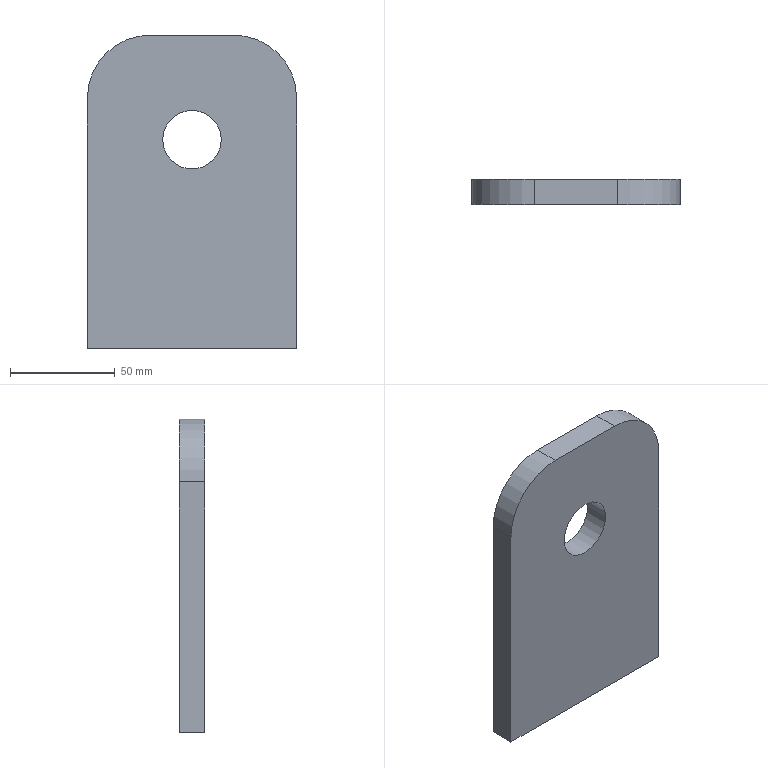Component | NX | CHAPA_GARAFA_2 | 1 solid | 9 faces | box 100 x 12 x 150 mm | volume 167976 mm3 | plane 6 | cylinder 3 | commonest cylinder face diameters 60 x2 28 x1
STEP:
#1=CARTESIAN_POINT('',(0.,0.,0.));
#2=DIRECTION('',(0.,0.,1.));
#3=DIRECTION('',(1.,0.,0.));
#4=AXIS2_PLACEMENT_3D('',#1,#2,#3);
#5=CARTESIAN_POINT('',(110.,-371.8,920.));
#6=VERTEX_POINT('',#5);
#7=CARTESIAN_POINT('',(110.,-371.8,800.));
#8=VERTEX_POINT('',#7);
#9=CARTESIAN_POINT('',(110.,-371.8,920.));
#10=DIRECTION('',(-0.,0.,-1.));
#11=VECTOR('',#10,1.);
#12=LINE('',#9,#11);
#13=CARTESIAN_POINT('',(110.,-359.8,920.));
#14=DIRECTION('',(-1.,0.,0.));
#15=DIRECTION('',(-0.,0.,-1.));
#16=AXIS2_PLACEMENT_3D('',#13,#14,#15);
#17=PLANE('',#16);
#18=CARTESIAN_POINT('',(0.,12.));
#19=DIRECTION('',(1.,0.));
#20=VECTOR('',#19,1.);
#21=LINE('',#18,#20);
#22=(GEOMETRIC_REPRESENTATION_CONTEXT(2)PARAMETRIC_REPRESENTATION_CONTEXT()REPRESENTATION_CONTEXT('',''));
#23=DEFINITIONAL_REPRESENTATION('',(#21),#22);
#24=PCURVE('',#17,#23);
#25=CARTESIAN_POINT('',(40.,-371.8,920.));
#26=DIRECTION('',(0.,1.,0.));
#27=DIRECTION('',(0.,0.,-1.));
#28=AXIS2_PLACEMENT_3D('',#25,#26,#27);
#29=PLANE('',#28);
#30=CARTESIAN_POINT('',(0.,-70.));
#31=DIRECTION('',(1.,0.));
#32=VECTOR('',#31,1.);
#33=LINE('',#30,#32);
#34=(GEOMETRIC_REPRESENTATION_CONTEXT(2)PARAMETRIC_REPRESENTATION_CONTEXT()REPRESENTATION_CONTEXT('',''));
#35=DEFINITIONAL_REPRESENTATION('',(#33),#34);
#36=PCURVE('',#29,#35);
#37=SURFACE_CURVE('',#12,(#24,#36),.PCURVE_S1.);
#38=EDGE_CURVE('',#6,#8,#37,.T.);
#39=ORIENTED_EDGE('',*,*,#38,.T.);
#40=CARTESIAN_POINT('',(110.,-359.8,800.));
#41=VERTEX_POINT('',#40);
#42=CARTESIAN_POINT('',(110.,-359.8,800.));
#43=DIRECTION('',(0.,-1.,0.));
#44=VECTOR('',#43,1.);
#45=LINE('',#42,#44);
#46=CARTESIAN_POINT('',(120.,0.));
#47=DIRECTION('',(0.,1.));
#48=VECTOR('',#47,1.);
#49=LINE('',#46,#48);
#50=(GEOMETRIC_REPRESENTATION_CONTEXT(2)PARAMETRIC_REPRESENTATION_CONTEXT()REPRESENTATION_CONTEXT('',''));
#51=DEFINITIONAL_REPRESENTATION('',(#49),#50);
#52=PCURVE('',#17,#51);
#53=CARTESIAN_POINT('',(110.,-359.8,800.));
#54=DIRECTION('',(0.,0.,1.));
#55=DIRECTION('',(-1.,0.,0.));
#56=AXIS2_PLACEMENT_3D('',#53,#54,#55);
#57=PLANE('',#56);
#58=CARTESIAN_POINT('',(0.,0.));
#59=DIRECTION('',(0.,1.));
#60=VECTOR('',#59,1.);
#61=LINE('',#58,#60);
#62=(GEOMETRIC_REPRESENTATION_CONTEXT(2)PARAMETRIC_REPRESENTATION_CONTEXT()REPRESENTATION_CONTEXT('',''));
#63=DEFINITIONAL_REPRESENTATION('',(#61),#62);
#64=PCURVE('',#57,#63);
#65=SURFACE_CURVE('',#45,(#52,#64),.PCURVE_S1.);
#66=EDGE_CURVE('',#41,#8,#65,.T.);
#67=ORIENTED_EDGE('',*,*,#66,.F.);
#68=CARTESIAN_POINT('',(110.,-359.8,920.));
#69=VERTEX_POINT('',#68);
#70=CARTESIAN_POINT('',(110.,-359.8,920.));
#71=DIRECTION('',(-0.,0.,-1.));
#72=VECTOR('',#71,1.);
#73=LINE('',#70,#72);
#74=CARTESIAN_POINT('',(0.,0.));
#75=DIRECTION('',(1.,0.));
#76=VECTOR('',#75,1.);
#77=LINE('',#74,#76);
#78=(GEOMETRIC_REPRESENTATION_CONTEXT(2)PARAMETRIC_REPRESENTATION_CONTEXT()REPRESENTATION_CONTEXT('',''));
#79=DEFINITIONAL_REPRESENTATION('',(#77),#78);
#80=PCURVE('',#17,#79);
#81=CARTESIAN_POINT('',(40.,-359.8,920.));
#82=DIRECTION('',(0.,1.,0.));
#83=DIRECTION('',(0.,0.,-1.));
#84=AXIS2_PLACEMENT_3D('',#81,#82,#83);
#85=PLANE('',#84);
#86=CARTESIAN_POINT('',(0.,-70.));
#87=DIRECTION('',(1.,0.));
#88=VECTOR('',#87,1.);
#89=LINE('',#86,#88);
#90=(GEOMETRIC_REPRESENTATION_CONTEXT(2)PARAMETRIC_REPRESENTATION_CONTEXT()REPRESENTATION_CONTEXT('',''));
#91=DEFINITIONAL_REPRESENTATION('',(#89),#90);
#92=PCURVE('',#85,#91);
#93=SURFACE_CURVE('',#73,(#80,#92),.PCURVE_S1.);
#94=EDGE_CURVE('',#69,#41,#93,.T.);
#95=ORIENTED_EDGE('',*,*,#94,.F.);
#96=CARTESIAN_POINT('',(110.,-359.8,920.));
#97=DIRECTION('',(0.,-1.,0.));
#98=VECTOR('',#97,1.);
#99=LINE('',#96,#98);
#100=CARTESIAN_POINT('',(0.,0.));
#101=DIRECTION('',(0.,1.));
#102=VECTOR('',#101,1.);
#103=LINE('',#100,#102);
#104=(GEOMETRIC_REPRESENTATION_CONTEXT(2)PARAMETRIC_REPRESENTATION_CONTEXT()REPRESENTATION_CONTEXT('',''));
#105=DEFINITIONAL_REPRESENTATION('',(#103),#104);
#106=PCURVE('',#17,#105);
#107=CARTESIAN_POINT('',(80.,-359.8,920.));
#108=DIRECTION('',(0.,-1.,0.));
#109=DIRECTION('',(0.,0.,1.));
#110=AXIS2_PLACEMENT_3D('',#107,#108,#109);
#111=CYLINDRICAL_SURFACE('',#110,30.);
#112=CARTESIAN_POINT('',(4.712,0.));
#113=DIRECTION('',(0.,1.));
#114=VECTOR('',#113,1.);
#115=LINE('',#112,#114);
#116=(GEOMETRIC_REPRESENTATION_CONTEXT(2)PARAMETRIC_REPRESENTATION_CONTEXT()REPRESENTATION_CONTEXT('',''));
#117=DEFINITIONAL_REPRESENTATION('',(#115),#116);
#118=PCURVE('',#111,#117);
#119=SURFACE_CURVE('',#99,(#106,#118),.PCURVE_S1.);
#120=EDGE_CURVE('',#69,#6,#119,.T.);
#121=ORIENTED_EDGE('',*,*,#120,.T.);
#122=EDGE_LOOP('',(#39,#67,#95,#121));
#123=FACE_BOUND('',#122,.T.);
#124=ADVANCED_FACE('',(#123),#17,.F.);
#125=CARTESIAN_POINT('',(10.,-371.8,800.));
#126=VERTEX_POINT('',#125);
#127=CARTESIAN_POINT('',(110.,-371.8,800.));
#128=DIRECTION('',(-1.,0.,0.));
#129=VECTOR('',#128,1.);
#130=LINE('',#127,#129);
#131=CARTESIAN_POINT('',(0.,12.));
#132=DIRECTION('',(1.,0.));
#133=VECTOR('',#132,1.);
#134=LINE('',#131,#133);
#135=(GEOMETRIC_REPRESENTATION_CONTEXT(2)PARAMETRIC_REPRESENTATION_CONTEXT()REPRESENTATION_CONTEXT('',''));
#136=DEFINITIONAL_REPRESENTATION('',(#134),#135);
#137=PCURVE('',#57,#136);
#138=CARTESIAN_POINT('',(120.,-70.));
#139=DIRECTION('',(-0.,1.));
#140=VECTOR('',#139,1.);
#141=LINE('',#138,#140);
#142=(GEOMETRIC_REPRESENTATION_CONTEXT(2)PARAMETRIC_REPRESENTATION_CONTEXT()REPRESENTATION_CONTEXT('',''));
#143=DEFINITIONAL_REPRESENTATION('',(#141),#142);
#144=PCURVE('',#29,#143);
#145=SURFACE_CURVE('',#130,(#137,#144),.PCURVE_S1.);
#146=EDGE_CURVE('',#8,#126,#145,.T.);
#147=ORIENTED_EDGE('',*,*,#146,.T.);
#148=CARTESIAN_POINT('',(10.,-359.8,800.));
#149=VERTEX_POINT('',#148);
#150=CARTESIAN_POINT('',(10.,-359.8,800.));
#151=DIRECTION('',(0.,-1.,0.));
#152=VECTOR('',#151,1.);
#153=LINE('',#150,#152);
#154=CARTESIAN_POINT('',(100.,0.));
#155=DIRECTION('',(0.,1.));
#156=VECTOR('',#155,1.);
#157=LINE('',#154,#156);
#158=(GEOMETRIC_REPRESENTATION_CONTEXT(2)PARAMETRIC_REPRESENTATION_CONTEXT()REPRESENTATION_CONTEXT('',''));
#159=DEFINITIONAL_REPRESENTATION('',(#157),#158);
#160=PCURVE('',#57,#159);
#161=CARTESIAN_POINT('',(10.,-359.8,800.));
#162=DIRECTION('',(1.,0.,0.));
#163=DIRECTION('',(0.,0.,1.));
#164=AXIS2_PLACEMENT_3D('',#161,#162,#163);
#165=PLANE('',#164);
#166=CARTESIAN_POINT('',(0.,0.));
#167=DIRECTION('',(0.,1.));
#168=VECTOR('',#167,1.);
#169=LINE('',#166,#168);
#170=(GEOMETRIC_REPRESENTATION_CONTEXT(2)PARAMETRIC_REPRESENTATION_CONTEXT()REPRESENTATION_CONTEXT('',''));
#171=DEFINITIONAL_REPRESENTATION('',(#169),#170);
#172=PCURVE('',#165,#171);
#173=SURFACE_CURVE('',#153,(#160,#172),.PCURVE_S1.);
#174=EDGE_CURVE('',#149,#126,#173,.T.);
#175=ORIENTED_EDGE('',*,*,#174,.F.);
#176=CARTESIAN_POINT('',(110.,-359.8,800.));
#177=DIRECTION('',(-1.,0.,0.));
#178=VECTOR('',#177,1.);
#179=LINE('',#176,#178);
#180=CARTESIAN_POINT('',(0.,0.));
#181=DIRECTION('',(1.,0.));
#182=VECTOR('',#181,1.);
#183=LINE('',#180,#182);
#184=(GEOMETRIC_REPRESENTATION_CONTEXT(2)PARAMETRIC_REPRESENTATION_CONTEXT()REPRESENTATION_CONTEXT('',''));
#185=DEFINITIONAL_REPRESENTATION('',(#183),#184);
#186=PCURVE('',#57,#185);
#187=CARTESIAN_POINT('',(120.,-70.));
#188=DIRECTION('',(-0.,1.));
#189=VECTOR('',#188,1.);
#190=LINE('',#187,#189);
#191=(GEOMETRIC_REPRESENTATION_CONTEXT(2)PARAMETRIC_REPRESENTATION_CONTEXT()REPRESENTATION_CONTEXT('',''));
#192=DEFINITIONAL_REPRESENTATION('',(#190),#191);
#193=PCURVE('',#85,#192);
#194=SURFACE_CURVE('',#179,(#186,#193),.PCURVE_S1.);
#195=EDGE_CURVE('',#41,#149,#194,.T.);
#196=ORIENTED_EDGE('',*,*,#195,.F.);
#197=ORIENTED_EDGE('',*,*,#66,.T.);
#198=EDGE_LOOP('',(#147,#175,#196,#197));
#199=FACE_BOUND('',#198,.T.);
#200=ADVANCED_FACE('',(#199),#57,.F.);
#201=CARTESIAN_POINT('',(10.,-371.8,920.));
#202=VERTEX_POINT('',#201);
#203=CARTESIAN_POINT('',(10.,-371.8,800.));
#204=DIRECTION('',(0.,0.,1.));
#205=VECTOR('',#204,1.);
#206=LINE('',#203,#205);
#207=CARTESIAN_POINT('',(0.,12.));
#208=DIRECTION('',(1.,0.));
#209=VECTOR('',#208,1.);
#210=LINE('',#207,#209);
#211=(GEOMETRIC_REPRESENTATION_CONTEXT(2)PARAMETRIC_REPRESENTATION_CONTEXT()REPRESENTATION_CONTEXT('',''));
#212=DEFINITIONAL_REPRESENTATION('',(#210),#211);
#213=PCURVE('',#165,#212);
#214=CARTESIAN_POINT('',(120.,30.));
#215=DIRECTION('',(-1.,0.));
#216=VECTOR('',#215,1.);
#217=LINE('',#214,#216);
#218=(GEOMETRIC_REPRESENTATION_CONTEXT(2)PARAMETRIC_REPRESENTATION_CONTEXT()REPRESENTATION_CONTEXT('',''));
#219=DEFINITIONAL_REPRESENTATION('',(#217),#218);
#220=PCURVE('',#29,#219);
#221=SURFACE_CURVE('',#206,(#213,#220),.PCURVE_S1.);
#222=EDGE_CURVE('',#126,#202,#221,.T.);
#223=ORIENTED_EDGE('',*,*,#222,.T.);
#224=CARTESIAN_POINT('',(10.,-359.8,920.));
#225=VERTEX_POINT('',#224);
#226=CARTESIAN_POINT('',(10.,-359.8,920.));
#227=DIRECTION('',(0.,-1.,0.));
#228=VECTOR('',#227,1.);
#229=LINE('',#226,#228);
#230=CARTESIAN_POINT('',(120.,0.));
#231=DIRECTION('',(0.,1.));
#232=VECTOR('',#231,1.);
#233=LINE('',#230,#232);
#234=(GEOMETRIC_REPRESENTATION_CONTEXT(2)PARAMETRIC_REPRESENTATION_CONTEXT()REPRESENTATION_CONTEXT('',''));
#235=DEFINITIONAL_REPRESENTATION('',(#233),#234);
#236=PCURVE('',#165,#235);
#237=CARTESIAN_POINT('',(40.,-359.8,920.));
#238=DIRECTION('',(0.,-1.,0.));
#239=DIRECTION('',(0.,0.,1.));
#240=AXIS2_PLACEMENT_3D('',#237,#238,#239);
#241=CYLINDRICAL_SURFACE('',#240,30.);
#242=CARTESIAN_POINT('',(1.571,0.));
#243=DIRECTION('',(0.,1.));
#244=VECTOR('',#243,1.);
#245=LINE('',#242,#244);
#246=(GEOMETRIC_REPRESENTATION_CONTEXT(2)PARAMETRIC_REPRESENTATION_CONTEXT()REPRESENTATION_CONTEXT('',''));
#247=DEFINITIONAL_REPRESENTATION('',(#245),#246);
#248=PCURVE('',#241,#247);
#249=SURFACE_CURVE('',#229,(#236,#248),.PCURVE_S1.);
#250=EDGE_CURVE('',#225,#202,#249,.T.);
#251=ORIENTED_EDGE('',*,*,#250,.F.);
#252=CARTESIAN_POINT('',(10.,-359.8,800.));
#253=DIRECTION('',(0.,0.,1.));
#254=VECTOR('',#253,1.);
#255=LINE('',#252,#254);
#256=CARTESIAN_POINT('',(0.,0.));
#257=DIRECTION('',(1.,0.));
#258=VECTOR('',#257,1.);
#259=LINE('',#256,#258);
#260=(GEOMETRIC_REPRESENTATION_CONTEXT(2)PARAMETRIC_REPRESENTATION_CONTEXT()REPRESENTATION_CONTEXT('',''));
#261=DEFINITIONAL_REPRESENTATION('',(#259),#260);
#262=PCURVE('',#165,#261);
#263=CARTESIAN_POINT('',(120.,30.));
#264=DIRECTION('',(-1.,0.));
#265=VECTOR('',#264,1.);
#266=LINE('',#263,#265);
#267=(GEOMETRIC_REPRESENTATION_CONTEXT(2)PARAMETRIC_REPRESENTATION_CONTEXT()REPRESENTATION_CONTEXT('',''));
#268=DEFINITIONAL_REPRESENTATION('',(#266),#267);
#269=PCURVE('',#85,#268);
#270=SURFACE_CURVE('',#255,(#262,#269),.PCURVE_S1.);
#271=EDGE_CURVE('',#149,#225,#270,.T.);
#272=ORIENTED_EDGE('',*,*,#271,.F.);
#273=ORIENTED_EDGE('',*,*,#174,.T.);
#274=EDGE_LOOP('',(#223,#251,#272,#273));
#275=FACE_BOUND('',#274,.T.);
#276=ADVANCED_FACE('',(#275),#165,.F.);
#277=CARTESIAN_POINT('',(40.,-371.8,950.));
#278=VERTEX_POINT('',#277);
#279=CARTESIAN_POINT('',(40.,-371.8,920.));
#280=DIRECTION('',(0.,1.,0.));
#281=DIRECTION('',(-1.,0.,0.));
#282=AXIS2_PLACEMENT_3D('',#279,#280,#281);
#283=CIRCLE('',#282,30.);
#284=CARTESIAN_POINT('',(1.571,12.));
#285=DIRECTION('',(-1.,0.));
#286=VECTOR('',#285,1.);
#287=LINE('',#284,#286);
#288=(GEOMETRIC_REPRESENTATION_CONTEXT(2)PARAMETRIC_REPRESENTATION_CONTEXT()REPRESENTATION_CONTEXT('',''));
#289=DEFINITIONAL_REPRESENTATION('',(#287),#288);
#290=PCURVE('',#241,#289);
#291=CARTESIAN_POINT('',(0.,0.));
#292=DIRECTION('',(0.,1.));
#293=AXIS2_PLACEMENT_2D('',#291,#292);
#294=CIRCLE('',#293,30.);
#295=(GEOMETRIC_REPRESENTATION_CONTEXT(2)PARAMETRIC_REPRESENTATION_CONTEXT()REPRESENTATION_CONTEXT('',''));
#296=DEFINITIONAL_REPRESENTATION('',(#294),#295);
#297=PCURVE('',#29,#296);
#298=SURFACE_CURVE('',#283,(#290,#297),.PCURVE_S1.);
#299=EDGE_CURVE('',#202,#278,#298,.T.);
#300=ORIENTED_EDGE('',*,*,#299,.T.);
#301=CARTESIAN_POINT('',(40.,-359.8,950.));
#302=VERTEX_POINT('',#301);
#303=CARTESIAN_POINT('',(40.,-359.8,950.));
#304=DIRECTION('',(0.,-1.,0.));
#305=VECTOR('',#304,1.);
#306=LINE('',#303,#305);
#307=CARTESIAN_POINT('',(0.,0.));
#308=DIRECTION('',(0.,1.));
#309=VECTOR('',#308,1.);
#310=LINE('',#307,#309);
#311=(GEOMETRIC_REPRESENTATION_CONTEXT(2)PARAMETRIC_REPRESENTATION_CONTEXT()REPRESENTATION_CONTEXT('',''));
#312=DEFINITIONAL_REPRESENTATION('',(#310),#311);
#313=PCURVE('',#241,#312);
#314=CARTESIAN_POINT('',(40.,-359.8,950.));
#315=DIRECTION('',(-0.,0.,-1.));
#316=DIRECTION('',(1.,0.,-0.));
#317=AXIS2_PLACEMENT_3D('',#314,#315,#316);
#318=PLANE('',#317);
#319=CARTESIAN_POINT('',(0.,0.));
#320=DIRECTION('',(0.,1.));
#321=VECTOR('',#320,1.);
#322=LINE('',#319,#321);
#323=(GEOMETRIC_REPRESENTATION_CONTEXT(2)PARAMETRIC_REPRESENTATION_CONTEXT()REPRESENTATION_CONTEXT('',''));
#324=DEFINITIONAL_REPRESENTATION('',(#322),#323);
#325=PCURVE('',#318,#324);
#326=SURFACE_CURVE('',#306,(#313,#325),.PCURVE_S1.);
#327=EDGE_CURVE('',#302,#278,#326,.T.);
#328=ORIENTED_EDGE('',*,*,#327,.F.);
#329=CARTESIAN_POINT('',(40.,-359.8,920.));
#330=DIRECTION('',(0.,1.,0.));
#331=DIRECTION('',(-1.,0.,0.));
#332=AXIS2_PLACEMENT_3D('',#329,#330,#331);
#333=CIRCLE('',#332,30.);
#334=CARTESIAN_POINT('',(1.571,0.));
#335=DIRECTION('',(-1.,0.));
#336=VECTOR('',#335,1.);
#337=LINE('',#334,#336);
#338=(GEOMETRIC_REPRESENTATION_CONTEXT(2)PARAMETRIC_REPRESENTATION_CONTEXT()REPRESENTATION_CONTEXT('',''));
#339=DEFINITIONAL_REPRESENTATION('',(#337),#338);
#340=PCURVE('',#241,#339);
#341=CARTESIAN_POINT('',(0.,0.));
#342=DIRECTION('',(0.,1.));
#343=AXIS2_PLACEMENT_2D('',#341,#342);
#344=CIRCLE('',#343,30.);
#345=(GEOMETRIC_REPRESENTATION_CONTEXT(2)PARAMETRIC_REPRESENTATION_CONTEXT()REPRESENTATION_CONTEXT('',''));
#346=DEFINITIONAL_REPRESENTATION('',(#344),#345);
#347=PCURVE('',#85,#346);
#348=SURFACE_CURVE('',#333,(#340,#347),.PCURVE_S1.);
#349=EDGE_CURVE('',#225,#302,#348,.T.);
#350=ORIENTED_EDGE('',*,*,#349,.F.);
#351=ORIENTED_EDGE('',*,*,#250,.T.);
#352=EDGE_LOOP('',(#300,#328,#350,#351));
#353=FACE_BOUND('',#352,.T.);
#354=ADVANCED_FACE('',(#353),#241,.T.);
#355=CARTESIAN_POINT('',(80.,-371.8,950.));
#356=VERTEX_POINT('',#355);
#357=CARTESIAN_POINT('',(40.,-371.8,950.));
#358=DIRECTION('',(1.,0.,-0.));
#359=VECTOR('',#358,1.);
#360=LINE('',#357,#359);
#361=CARTESIAN_POINT('',(0.,12.));
#362=DIRECTION('',(1.,0.));
#363=VECTOR('',#362,1.);
#364=LINE('',#361,#363);
#365=(GEOMETRIC_REPRESENTATION_CONTEXT(2)PARAMETRIC_REPRESENTATION_CONTEXT()REPRESENTATION_CONTEXT('',''));
#366=DEFINITIONAL_REPRESENTATION('',(#364),#365);
#367=PCURVE('',#318,#366);
#368=CARTESIAN_POINT('',(-30.,0.));
#369=DIRECTION('',(0.,-1.));
#370=VECTOR('',#369,1.);
#371=LINE('',#368,#370);
#372=(GEOMETRIC_REPRESENTATION_CONTEXT(2)PARAMETRIC_REPRESENTATION_CONTEXT()REPRESENTATION_CONTEXT('',''));
#373=DEFINITIONAL_REPRESENTATION('',(#371),#372);
#374=PCURVE('',#29,#373);
#375=SURFACE_CURVE('',#360,(#367,#374),.PCURVE_S1.);
#376=EDGE_CURVE('',#278,#356,#375,.T.);
#377=ORIENTED_EDGE('',*,*,#376,.T.);
#378=CARTESIAN_POINT('',(80.,-359.8,950.));
#379=VERTEX_POINT('',#378);
#380=CARTESIAN_POINT('',(80.,-359.8,950.));
#381=DIRECTION('',(0.,-1.,0.));
#382=VECTOR('',#381,1.);
#383=LINE('',#380,#382);
#384=CARTESIAN_POINT('',(40.,0.));
#385=DIRECTION('',(0.,1.));
#386=VECTOR('',#385,1.);
#387=LINE('',#384,#386);
#388=(GEOMETRIC_REPRESENTATION_CONTEXT(2)PARAMETRIC_REPRESENTATION_CONTEXT()REPRESENTATION_CONTEXT('',''));
#389=DEFINITIONAL_REPRESENTATION('',(#387),#388);
#390=PCURVE('',#318,#389);
#391=CARTESIAN_POINT('',(6.283,0.));
#392=DIRECTION('',(0.,1.));
#393=VECTOR('',#392,1.);
#394=LINE('',#391,#393);
#395=(GEOMETRIC_REPRESENTATION_CONTEXT(2)PARAMETRIC_REPRESENTATION_CONTEXT()REPRESENTATION_CONTEXT('',''));
#396=DEFINITIONAL_REPRESENTATION('',(#394),#395);
#397=PCURVE('',#111,#396);
#398=SURFACE_CURVE('',#383,(#390,#397),.PCURVE_S1.);
#399=EDGE_CURVE('',#379,#356,#398,.T.);
#400=ORIENTED_EDGE('',*,*,#399,.F.);
#401=CARTESIAN_POINT('',(40.,-359.8,950.));
#402=DIRECTION('',(1.,0.,-0.));
#403=VECTOR('',#402,1.);
#404=LINE('',#401,#403);
#405=CARTESIAN_POINT('',(0.,0.));
#406=DIRECTION('',(1.,0.));
#407=VECTOR('',#406,1.);
#408=LINE('',#405,#407);
#409=(GEOMETRIC_REPRESENTATION_CONTEXT(2)PARAMETRIC_REPRESENTATION_CONTEXT()REPRESENTATION_CONTEXT('',''));
#410=DEFINITIONAL_REPRESENTATION('',(#408),#409);
#411=PCURVE('',#318,#410);
#412=CARTESIAN_POINT('',(-30.,0.));
#413=DIRECTION('',(0.,-1.));
#414=VECTOR('',#413,1.);
#415=LINE('',#412,#414);
#416=(GEOMETRIC_REPRESENTATION_CONTEXT(2)PARAMETRIC_REPRESENTATION_CONTEXT()REPRESENTATION_CONTEXT('',''));
#417=DEFINITIONAL_REPRESENTATION('',(#415),#416);
#418=PCURVE('',#85,#417);
#419=SURFACE_CURVE('',#404,(#411,#418),.PCURVE_S1.);
#420=EDGE_CURVE('',#302,#379,#419,.T.);
#421=ORIENTED_EDGE('',*,*,#420,.F.);
#422=ORIENTED_EDGE('',*,*,#327,.T.);
#423=EDGE_LOOP('',(#377,#400,#421,#422));
#424=FACE_BOUND('',#423,.T.);
#425=ADVANCED_FACE('',(#424),#318,.F.);
#426=CARTESIAN_POINT('',(80.,-371.8,920.));
#427=DIRECTION('',(0.,1.,0.));
#428=DIRECTION('',(-1.,0.,0.));
#429=AXIS2_PLACEMENT_3D('',#426,#427,#428);
#430=CIRCLE('',#429,30.);
#431=CARTESIAN_POINT('',(7.854,12.));
#432=DIRECTION('',(-1.,0.));
#433=VECTOR('',#432,1.);
#434=LINE('',#431,#433);
#435=(GEOMETRIC_REPRESENTATION_CONTEXT(2)PARAMETRIC_REPRESENTATION_CONTEXT()REPRESENTATION_CONTEXT('',''));
#436=DEFINITIONAL_REPRESENTATION('',(#434),#435);
#437=PCURVE('',#111,#436);
#438=CARTESIAN_POINT('',(0.,-40.));
#439=DIRECTION('',(0.,1.));
#440=AXIS2_PLACEMENT_2D('',#438,#439);
#441=CIRCLE('',#440,30.);
#442=(GEOMETRIC_REPRESENTATION_CONTEXT(2)PARAMETRIC_REPRESENTATION_CONTEXT()REPRESENTATION_CONTEXT('',''));
#443=DEFINITIONAL_REPRESENTATION('',(#441),#442);
#444=PCURVE('',#29,#443);
#445=SURFACE_CURVE('',#430,(#437,#444),.PCURVE_S1.);
#446=EDGE_CURVE('',#356,#6,#445,.T.);
#447=ORIENTED_EDGE('',*,*,#446,.T.);
#448=ORIENTED_EDGE('',*,*,#120,.F.);
#449=CARTESIAN_POINT('',(80.,-359.8,920.));
#450=DIRECTION('',(0.,1.,0.));
#451=DIRECTION('',(-1.,0.,0.));
#452=AXIS2_PLACEMENT_3D('',#449,#450,#451);
#453=CIRCLE('',#452,30.);
#454=CARTESIAN_POINT('',(7.854,0.));
#455=DIRECTION('',(-1.,0.));
#456=VECTOR('',#455,1.);
#457=LINE('',#454,#456);
#458=(GEOMETRIC_REPRESENTATION_CONTEXT(2)PARAMETRIC_REPRESENTATION_CONTEXT()REPRESENTATION_CONTEXT('',''));
#459=DEFINITIONAL_REPRESENTATION('',(#457),#458);
#460=PCURVE('',#111,#459);
#461=CARTESIAN_POINT('',(0.,-40.));
#462=DIRECTION('',(0.,1.));
#463=AXIS2_PLACEMENT_2D('',#461,#462);
#464=CIRCLE('',#463,30.);
#465=(GEOMETRIC_REPRESENTATION_CONTEXT(2)PARAMETRIC_REPRESENTATION_CONTEXT()REPRESENTATION_CONTEXT('',''));
#466=DEFINITIONAL_REPRESENTATION('',(#464),#465);
#467=PCURVE('',#85,#466);
#468=SURFACE_CURVE('',#453,(#460,#467),.PCURVE_S1.);
#469=EDGE_CURVE('',#379,#69,#468,.T.);
#470=ORIENTED_EDGE('',*,*,#469,.F.);
#471=ORIENTED_EDGE('',*,*,#399,.T.);
#472=EDGE_LOOP('',(#447,#448,#470,#471));
#473=FACE_BOUND('',#472,.T.);
#474=ADVANCED_FACE('',(#473),#111,.T.);
#475=CARTESIAN_POINT('',(46.,-359.8,900.));
#476=VERTEX_POINT('',#475);
#477=CARTESIAN_POINT('',(60.,-359.8,900.));
#478=DIRECTION('',(0.,1.,0.));
#479=DIRECTION('',(-1.,0.,0.));
#480=AXIS2_PLACEMENT_3D('',#477,#478,#479);
#481=CIRCLE('',#480,14.);
#482=CARTESIAN_POINT('',(60.,-359.8,900.));
#483=DIRECTION('',(0.,-1.,0.));
#484=DIRECTION('',(0.,0.,1.));
#485=AXIS2_PLACEMENT_3D('',#482,#483,#484);
#486=CYLINDRICAL_SURFACE('',#485,14.);
#487=CARTESIAN_POINT('',(7.854,0.));
#488=DIRECTION('',(-1.,0.));
#489=VECTOR('',#488,1.);
#490=LINE('',#487,#489);
#491=(GEOMETRIC_REPRESENTATION_CONTEXT(2)PARAMETRIC_REPRESENTATION_CONTEXT()REPRESENTATION_CONTEXT('',''));
#492=DEFINITIONAL_REPRESENTATION('',(#490),#491);
#493=PCURVE('',#486,#492);
#494=CARTESIAN_POINT('',(20.,-20.));
#495=DIRECTION('',(0.,1.));
#496=AXIS2_PLACEMENT_2D('',#494,#495);
#497=CIRCLE('',#496,14.);
#498=(GEOMETRIC_REPRESENTATION_CONTEXT(2)PARAMETRIC_REPRESENTATION_CONTEXT()REPRESENTATION_CONTEXT('',''));
#499=DEFINITIONAL_REPRESENTATION('',(#497),#498);
#500=PCURVE('',#85,#499);
#501=SURFACE_CURVE('',#481,(#493,#500),.PCURVE_S1.);
#502=EDGE_CURVE('',#476,#476,#501,.T.);
#503=ORIENTED_EDGE('',*,*,#502,.F.);
#504=CARTESIAN_POINT('',(46.,-371.8,900.));
#505=VERTEX_POINT('',#504);
#506=CARTESIAN_POINT('',(46.,-359.8,900.));
#507=CARTESIAN_POINT('',(46.,-371.8,900.));
#508=B_SPLINE_CURVE_WITH_KNOTS('',1,(#506,#507),.UNSPECIFIED.,.F.,.F.,(2,2),(0.,12.),.PIECEWISE_BEZIER_KNOTS.);
#509=CARTESIAN_POINT('',(7.854,0.));
#510=DIRECTION('',(0.,1.));
#511=VECTOR('',#510,1.);
#512=LINE('',#509,#511);
#513=(GEOMETRIC_REPRESENTATION_CONTEXT(2)PARAMETRIC_REPRESENTATION_CONTEXT()REPRESENTATION_CONTEXT('',''));
#514=DEFINITIONAL_REPRESENTATION('',(#512),#513);
#515=PCURVE('',#486,#514);
#516=CARTESIAN_POINT('',(1.571,0.));
#517=DIRECTION('',(0.,1.));
#518=VECTOR('',#517,1.);
#519=LINE('',#516,#518);
#520=(GEOMETRIC_REPRESENTATION_CONTEXT(2)PARAMETRIC_REPRESENTATION_CONTEXT()REPRESENTATION_CONTEXT('',''));
#521=DEFINITIONAL_REPRESENTATION('',(#519),#520);
#522=PCURVE('',#486,#521);
#523=SEAM_CURVE('',#508,(#515,#522),.PCURVE_S1.);
#524=EDGE_CURVE('',#476,#505,#523,.T.);
#525=ORIENTED_EDGE('',*,*,#524,.T.);
#526=CARTESIAN_POINT('',(60.,-371.8,900.));
#527=DIRECTION('',(0.,1.,0.));
#528=DIRECTION('',(-1.,0.,0.));
#529=AXIS2_PLACEMENT_3D('',#526,#527,#528);
#530=CIRCLE('',#529,14.);
#531=CARTESIAN_POINT('',(7.854,12.));
#532=DIRECTION('',(-1.,0.));
#533=VECTOR('',#532,1.);
#534=LINE('',#531,#533);
#535=(GEOMETRIC_REPRESENTATION_CONTEXT(2)PARAMETRIC_REPRESENTATION_CONTEXT()REPRESENTATION_CONTEXT('',''));
#536=DEFINITIONAL_REPRESENTATION('',(#534),#535);
#537=PCURVE('',#486,#536);
#538=CARTESIAN_POINT('',(20.,-20.));
#539=DIRECTION('',(0.,1.));
#540=AXIS2_PLACEMENT_2D('',#538,#539);
#541=CIRCLE('',#540,14.);
#542=(GEOMETRIC_REPRESENTATION_CONTEXT(2)PARAMETRIC_REPRESENTATION_CONTEXT()REPRESENTATION_CONTEXT('',''));
#543=DEFINITIONAL_REPRESENTATION('',(#541),#542);
#544=PCURVE('',#29,#543);
#545=SURFACE_CURVE('',#530,(#537,#544),.PCURVE_S1.);
#546=EDGE_CURVE('',#505,#505,#545,.T.);
#547=ORIENTED_EDGE('',*,*,#546,.T.);
#548=ORIENTED_EDGE('',*,*,#524,.F.);
#549=EDGE_LOOP('',(#503,#525,#547,#548));
#550=FACE_BOUND('',#549,.F.);
#551=ADVANCED_FACE('',(#550),#486,.F.);
#552=ORIENTED_EDGE('',*,*,#94,.T.);
#553=ORIENTED_EDGE('',*,*,#195,.T.);
#554=ORIENTED_EDGE('',*,*,#271,.T.);
#555=ORIENTED_EDGE('',*,*,#349,.T.);
#556=ORIENTED_EDGE('',*,*,#420,.T.);
#557=ORIENTED_EDGE('',*,*,#469,.T.);
#558=EDGE_LOOP('',(#552,#553,#554,#555,#556,#557));
#559=FACE_BOUND('',#558,.T.);
#560=ORIENTED_EDGE('',*,*,#502,.F.);
#561=EDGE_LOOP('',(#560));
#562=FACE_BOUND('',#561,.T.);
#563=ADVANCED_FACE('',(#559,#562),#85,.T.);
#564=ORIENTED_EDGE('',*,*,#38,.F.);
#565=ORIENTED_EDGE('',*,*,#446,.F.);
#566=ORIENTED_EDGE('',*,*,#376,.F.);
#567=ORIENTED_EDGE('',*,*,#299,.F.);
#568=ORIENTED_EDGE('',*,*,#222,.F.);
#569=ORIENTED_EDGE('',*,*,#146,.F.);
#570=EDGE_LOOP('',(#564,#565,#566,#567,#568,#569));
#571=FACE_BOUND('',#570,.T.);
#572=ORIENTED_EDGE('',*,*,#546,.T.);
#573=EDGE_LOOP('',(#572));
#574=FACE_BOUND('',#573,.T.);
#575=ADVANCED_FACE('',(#571,#574),#29,.F.);
#576=CLOSED_SHELL('',(#124,#200,#276,#354,#425,#474,#551,#563,#575));
#577=MANIFOLD_SOLID_BREP('',#576);
#578=(LENGTH_UNIT()NAMED_UNIT(*)SI_UNIT(.MILLI.,.METRE.));
#579=UNCERTAINTY_MEASURE_WITH_UNIT(LENGTH_MEASURE(0.000001),#578,'','');
#580=(NAMED_UNIT(*)PLANE_ANGLE_UNIT()SI_UNIT($,.RADIAN.));
#581=(NAMED_UNIT(*)SI_UNIT($,.STERADIAN.)SOLID_ANGLE_UNIT());
#582=(GEOMETRIC_REPRESENTATION_CONTEXT(3)GLOBAL_UNCERTAINTY_ASSIGNED_CONTEXT((#579))GLOBAL_UNIT_ASSIGNED_CONTEXT((#578,#580,#581))REPRESENTATION_CONTEXT('',''));
#583=ADVANCED_BREP_SHAPE_REPRESENTATION('',(#4,#577),#582);